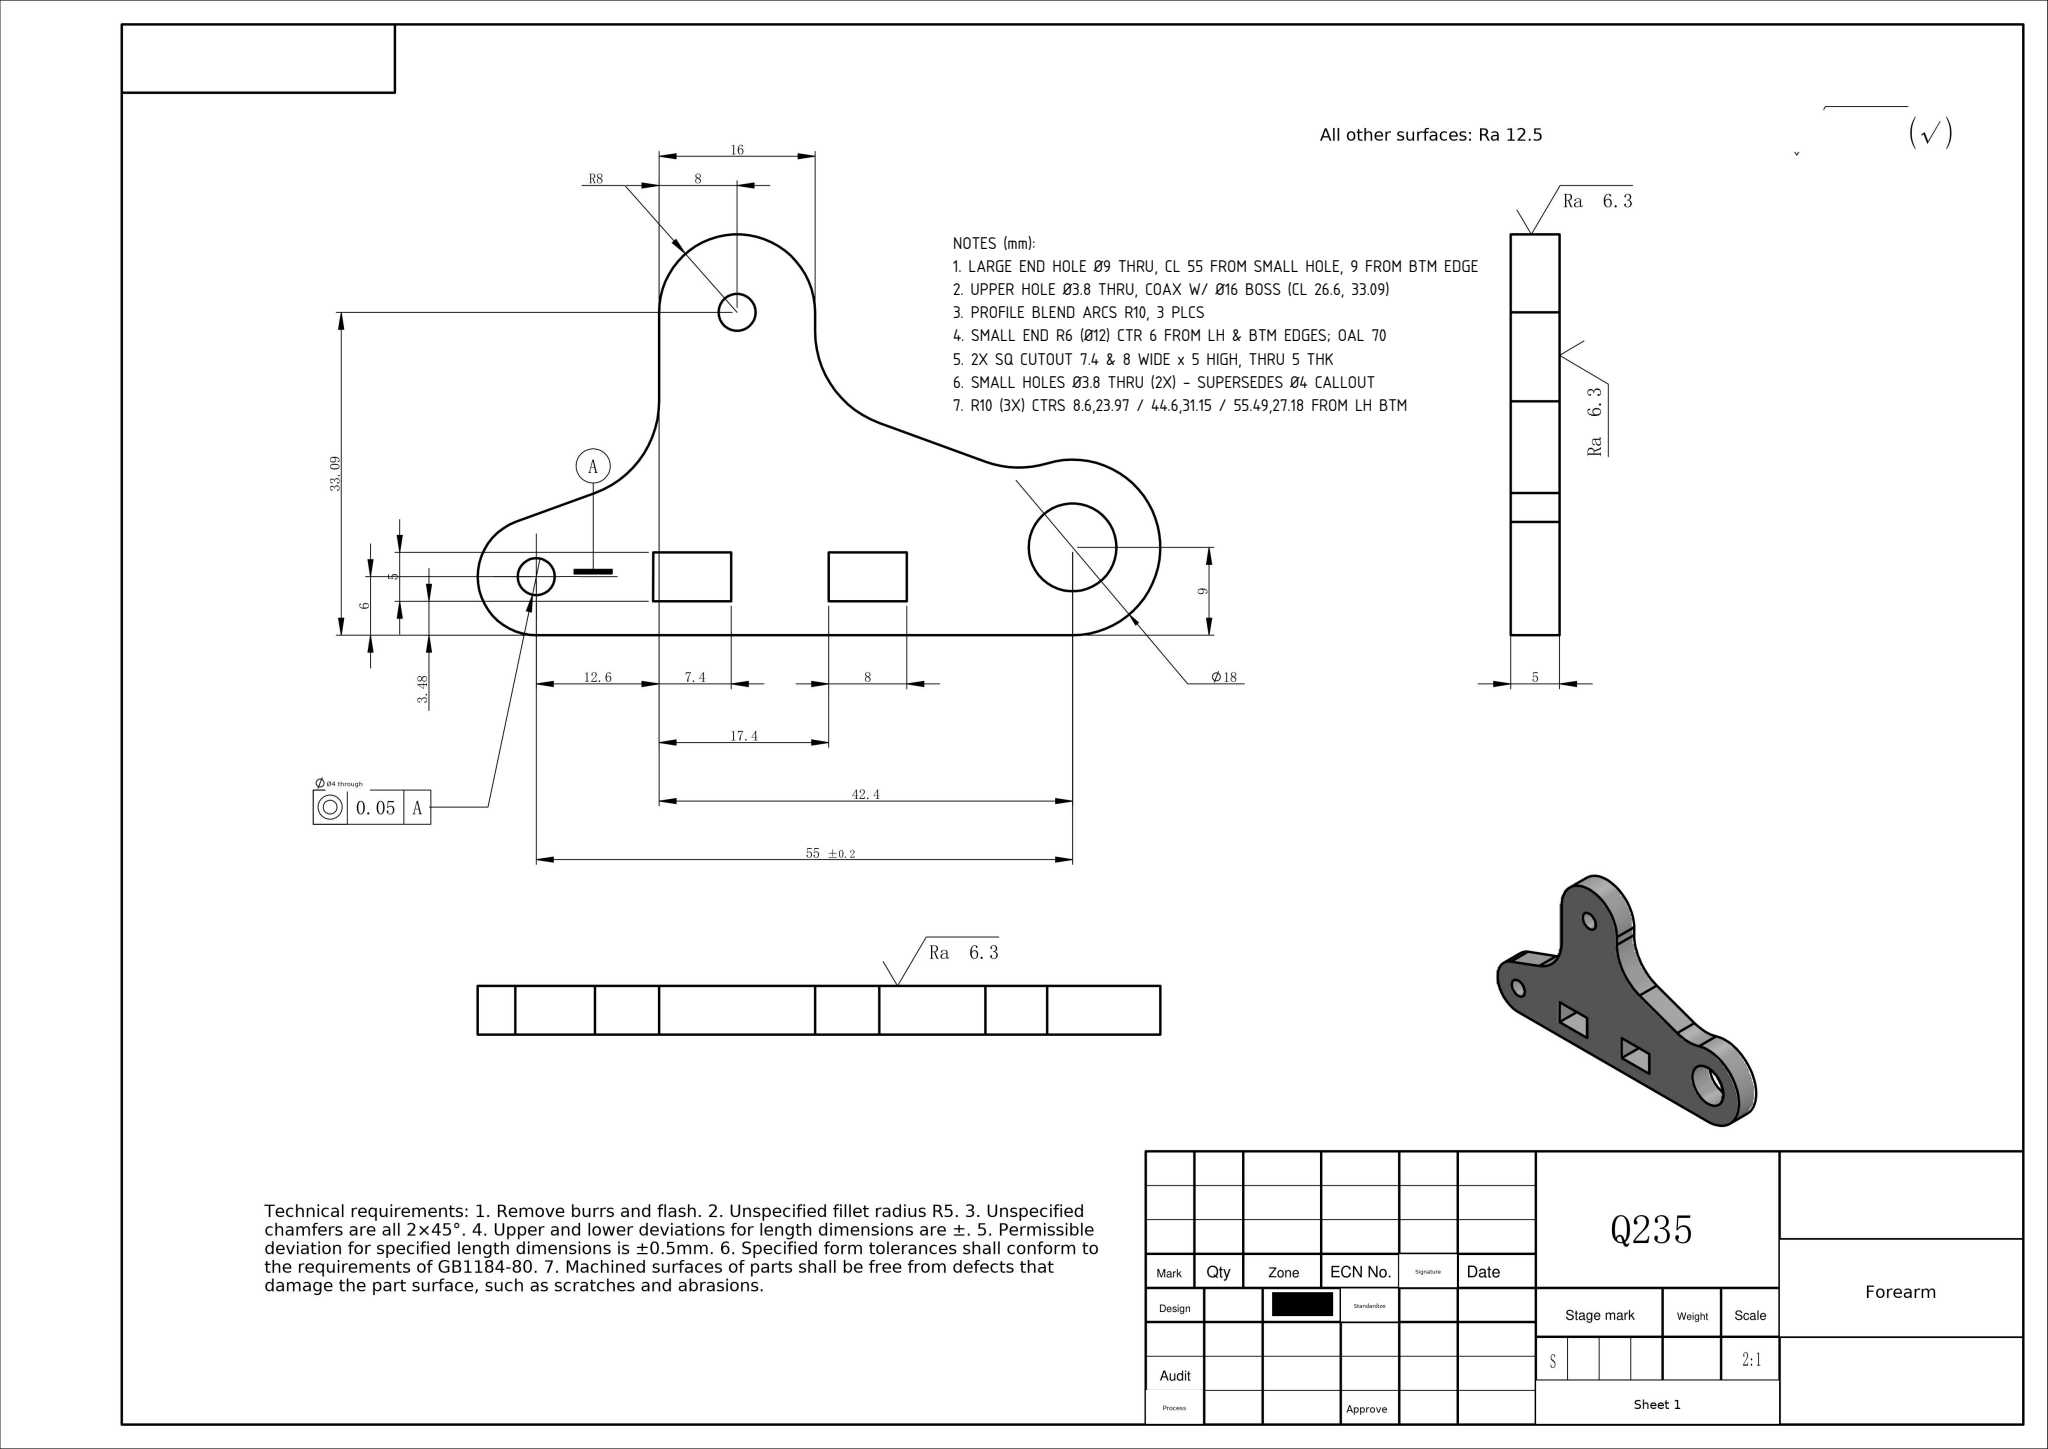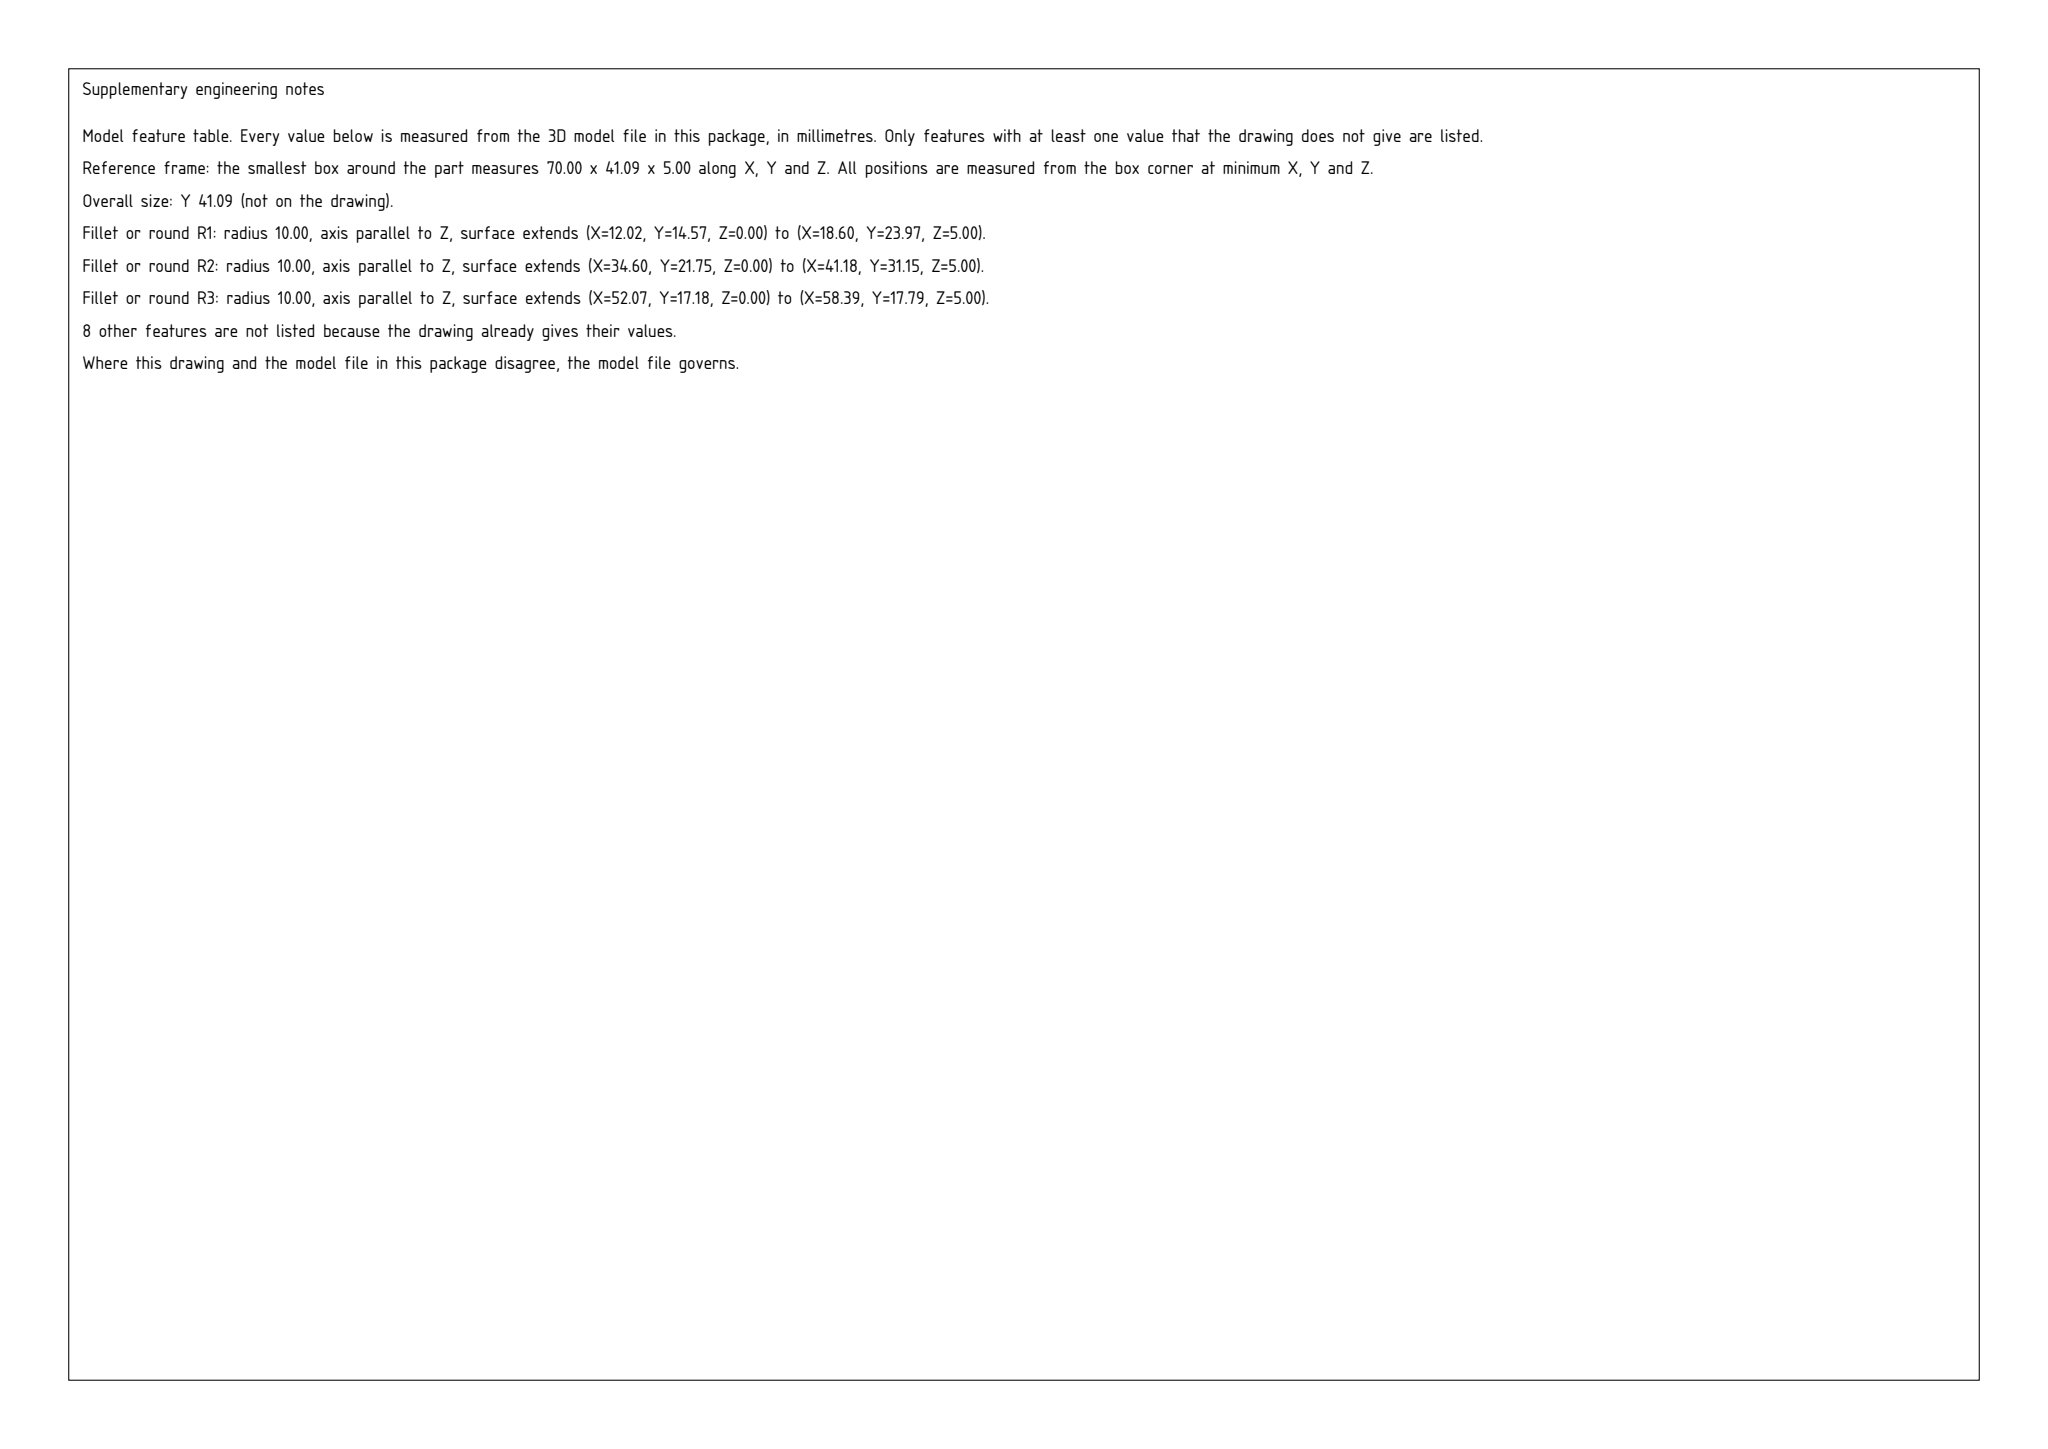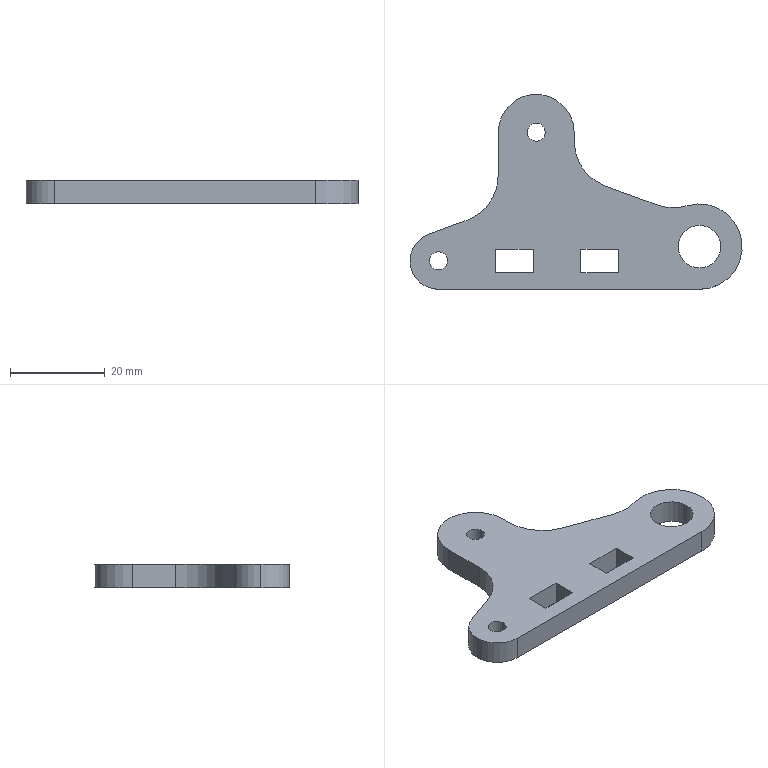Part | SolidWorks | mm | 1 solid | 28 faces | box 70 x 41.09 x 5 mm | volume 6865 mm3 | plane 15 | cylinder 13 | commonest cylinder face diameters 3.8 x4 20 x3 9 x2 12 x2 18 x1 16 x1
Drawing notes:
LARGE END HOLE Ø9 THRU, CL 55 FROM SMALL HOLE, 9 FROM BTM EDGE | from the solid: cylinder dia 9.0 axis z at (61.0,9.0), length 5.0 (thru 5 thk); coaxial with Ø18 boss; small hole CL at x=6 -> 55 apart
UPPER HOLE Ø3.8 THRU, COAX W/ Ø16 BOSS (CL 26.6, 33.09) | from the solid: cylinder dia 3.8 axis z at (26.6,33.09), length 5.0; Ø16 boss same CL
PROFILE BLEND ARCS R10, 3 PLCS | from the solid: three cylinders dia 20.0 axis z at (8.6,23.97), (44.6,31.15), (55.49,27.18) = R10
SMALL END R6 (Ø12) CTR 6 FROM LH & BTM EDGES; OAL 70 | from the solid: cyl Ø12 z-axis at (6,6); bbox_xyz x=70
2X SQ CUTOUT 7.4 & 8 WIDE x 5 HIGH, THRU 5 THK | from the solid: x planes 18.6/26.0 & 36.0/44.0; y planes 3.48/8.48; bbox z=5
SMALL HOLES Ø3.8 THRU (2X) - SUPERSEDES Ø4 CALLOUT | from the solid: cyl Ø3.8 z-axis at (6,6) and (26.6,33.09), length 5
R10 (3X) CTRS 8.6,23.97 / 44.6,31.15 / 55.49,27.18 FROM LH BTM | from the solid: Ø20 z-cyls at (8.6,23.97), (44.6,31.15), (55.49,27.18)
build123d program:
from build123d import *

# Parameters (mm, degrees)
ESQUISSE1_R        = 1.9
ESQUISSE1_R_2      = 4.5
ESQUISSE1_W        = 8
ESQUISSE1_H        = 5
BOSS_EXTRU_1_DEPTH = 5


with BuildPart() as part:
    # Esquisse1 → Boss.-Extru.1 (new body)
    with BuildSketch(Plane.XY):
        with BuildLine():
            Line((-22.984, -5.97), (-31.146, -8.942))
            ThreePointArc((-31.146, -8.942), (-34.9, -15.636), (-29, -20.545))
            Line((-29, -20.545), (26, -20.545))
            ThreePointArc((26, -20.545), (34.903, -10.225), (23.388, -2.932))
            ThreePointArc((23.388, -2.932), (20.213, -3.359), (17.066, -2.759))
            Line((17.066, -2.759), (6.175, 1.205))
            ThreePointArc((6.175, 1.205), (1.404, 4.866), (-0.4044, 10.602))
            Line((-0.4044, 10.602), (-0.4044, 12.545))
            ThreePointArc((-0.4044, 12.545), (-8.404, 20.545), (-16.404, 12.545))
            Line((-16.404, 12.545), (-16.404, 3.427))
            ThreePointArc((-16.404, 3.427), (-18.213, -2.309), (-22.984, -5.97))
        make_face()
        with Locations((-8.404, 12.545)):
            Circle(ESQUISSE1_R, mode=Mode.SUBTRACT)
        with Locations((-29, -14.545)):
            Circle(ESQUISSE1_R, mode=Mode.SUBTRACT)
        with Locations((26, -11.545)):
            Circle(ESQUISSE1_R_2, mode=Mode.SUBTRACT)
        with Locations((5, -14.565)):
            Rectangle(ESQUISSE1_W, ESQUISSE1_H, mode=Mode.SUBTRACT)
        Polygon((-17, -12.065), (-17.014, -17.065), (-9, -17.065), (-9, -12.065), align=None, mode=Mode.SUBTRACT)
    extrude(amount=BOSS_EXTRU_1_DEPTH)


solid = part.part